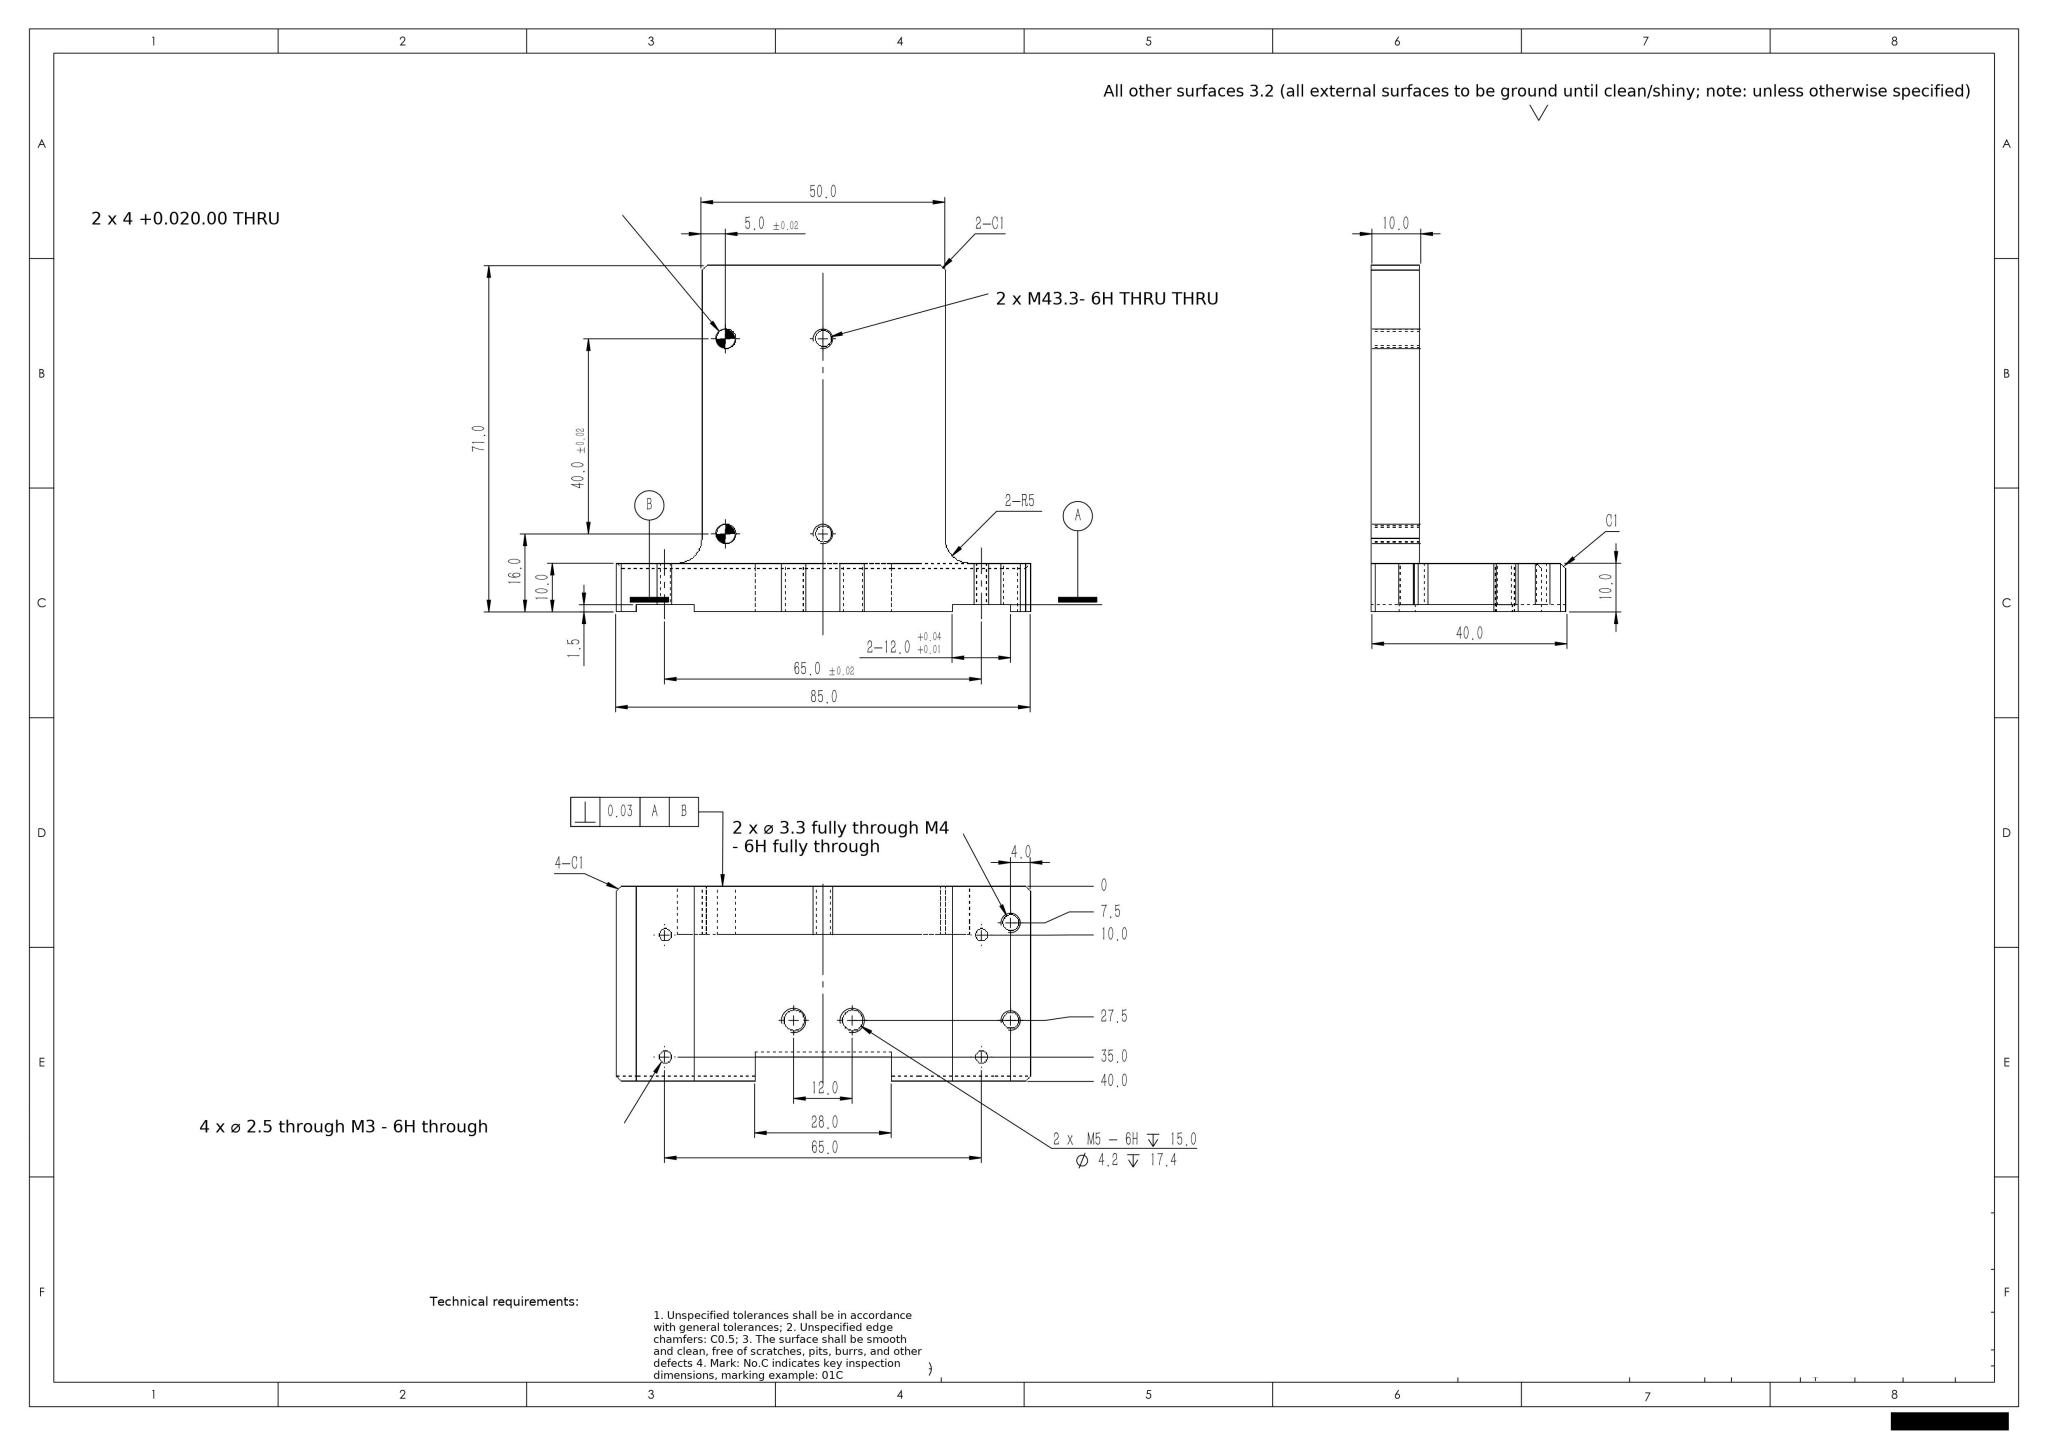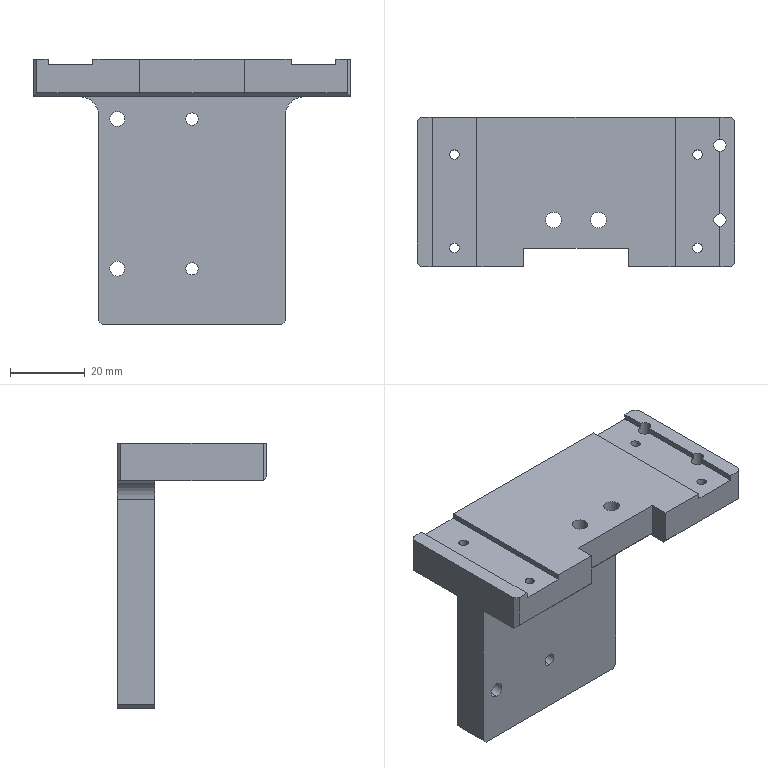Part | SolidWorks | mm | 1 solid | 59 faces | box 85 x 40 x 71 mm | volume 60671 mm3 | plane 33 | cylinder 26 | commonest cylinder face diameters 3.3 x8 2.5 x8 4.2 x4 4 x4 10 x2
build123d program:
from build123d import *

# Parameters (mm, degrees)
SKETCH1_W                  = 50
SKETCH1_H                  = 71
BOSS_EXTRUDE1_DEPTH        = 10
SKETCH18_W                 = 85
SKETCH18_H                 = 40
BOSS_EXTRUDE2_DEPTH        = 10
SKETCH2_W                  = 12
SKETCH2_H                  = 40
CUT_EXTRUDE1_DEPTH         = 1.5
M3_TAPPED_HOLE1_D          = 2.5
M4_TAPPED_HOLE1_D          = 3.3
SIZE_MM_DOWEL_PIN_HOLE_2_D = 4
SKETCH21_W                 = 28
SKETCH21_H                 = 15.122
CUT_EXTRUDE2_DEPTH         = 81.17
M5_TAPPED_HOLE1_D          = 4.2
M5_TAPPED_HOLE1_DEPTH      = 17.4
M5_TAPPED_HOLE1_TIP        = 1.262
M4_TAPPED_HOLE2_D          = 3.3
FILLET1_R                  = 5
CHAMFER1_SIZE              = 1


with BuildPart() as part:
    # Sketch1 → Boss-Extrude1 (new body)
    with BuildSketch(Plane(origin=(0, 0, 0), x_dir=(1, 0, 0), z_dir=(0, 1, 0))):
        Rectangle(SKETCH1_W, SKETCH1_H)
    extrude(amount=BOSS_EXTRUDE1_DEPTH)

    # Sketch18 → Boss-Extrude2 (add)
    with BuildSketch(Plane.XY.offset(35.5)):
        with Locations((0, -10)):
            Rectangle(SKETCH18_W, SKETCH18_H)
    extrude(amount=-BOSS_EXTRUDE2_DEPTH)

    # Sketch2 → Cut-Extrude1 (cut)
    with BuildSketch(Plane(origin=(0, -35, 35.5), x_dir=(1, 0, 0), z_dir=(0, 0, -1))):
        with Locations((32.5, -25)):
            Rectangle(SKETCH2_W, SKETCH2_H)
        with Locations((-32.5, -25)):
            Rectangle(SKETCH2_W, SKETCH2_H)
    extrude(amount=CUT_EXTRUDE1_DEPTH, mode=Mode.SUBTRACT)

    # M3 Tapped Hole1 (through all)
    with Locations(Plane(origin=(0, -25, 35.5), x_dir=(1, 0, 0), z_dir=(0, 0, 1))):
        with Locations((32.5, 25), (32.5, 0), (-32.5, 0), (-32.5, 25)):
            Hole(M3_TAPPED_HOLE1_D / 2)

    # M4 Tapped Hole1 (through all)
    with Locations(Plane(origin=(0, 10, 0), x_dir=(1, 0, 0), z_dir=(0, 1, 0))):
        with Locations((0, 20.5), (0, -19.5)):
            Hole(M4_TAPPED_HOLE1_D / 2)

    # Size mm Dowel Pin Hole 2 (through all)
    with Locations(Plane(origin=(0, 10, 0), x_dir=(1, 0, 0), z_dir=(0, 1, 0))):
        with Locations((-20, -19.5), (-20, 20.5)):
            Hole(SIZE_MM_DOWEL_PIN_HOLE_2_D / 2)

    # Sketch21 → Cut-Extrude2 (cut, through all)
    with BuildSketch(Plane(origin=(0, 0, 25.5), x_dir=(-1, 0, 0), z_dir=(0, 0, -1))):
        with Locations((0, -32.561)):
            Rectangle(SKETCH21_W, SKETCH21_H)
    extrude(amount=-CUT_EXTRUDE2_DEPTH, mode=Mode.SUBTRACT)

    # M5 Tapped Hole1
    with Locations(Plane(origin=(0, -50, 25.5), x_dir=(-1, 0, 0), z_dir=(0, 0, -1))):
        with Locations((-6, 32.5), (6, 32.5)):
            Hole(M5_TAPPED_HOLE1_D / 2, depth=M5_TAPPED_HOLE1_DEPTH)
            with Locations((0, 0, -(M5_TAPPED_HOLE1_DEPTH + M5_TAPPED_HOLE1_TIP / 2))):  # 118° drill point
                Cone(0, M5_TAPPED_HOLE1_D / 2, M5_TAPPED_HOLE1_TIP, mode=Mode.SUBTRACT)

    # M4 Tapped Hole2 (through all)
    with Locations(Plane(origin=(0, 0, 25.5), x_dir=(-1, 0, 0), z_dir=(0, 0, -1))):
        with Locations((-38.5, 2.5), (-38.5, -17.5)):
            Hole(M4_TAPPED_HOLE2_D / 2)

    # Fillet1
    fillet1_edges = [part.edges().sort_by_distance(p)[0] for p in [
        (25, 5, 25.5),
        (-25, 5, 25.5),
    ]]
    fillet(fillet1_edges, radius=FILLET1_R)

    # Chamfer1
    chamfer1_edges = [part.edges().sort_by_distance(p)[0] for p in [
        (28.25, -30, 25.5),
        (0, -25, 25.5),
        (-42.5, 10, 30.5),
        (-42.5, -30, 30.5),
        (42.5, 10, 30.5),
        (-28.25, -30, 25.5),
        (42.5, -30, 30.5),
        (-25, 5, -35.5),
        (25, 5, -35.5),
    ]]
    chamfer(chamfer1_edges, length=CHAMFER1_SIZE)


solid = part.part